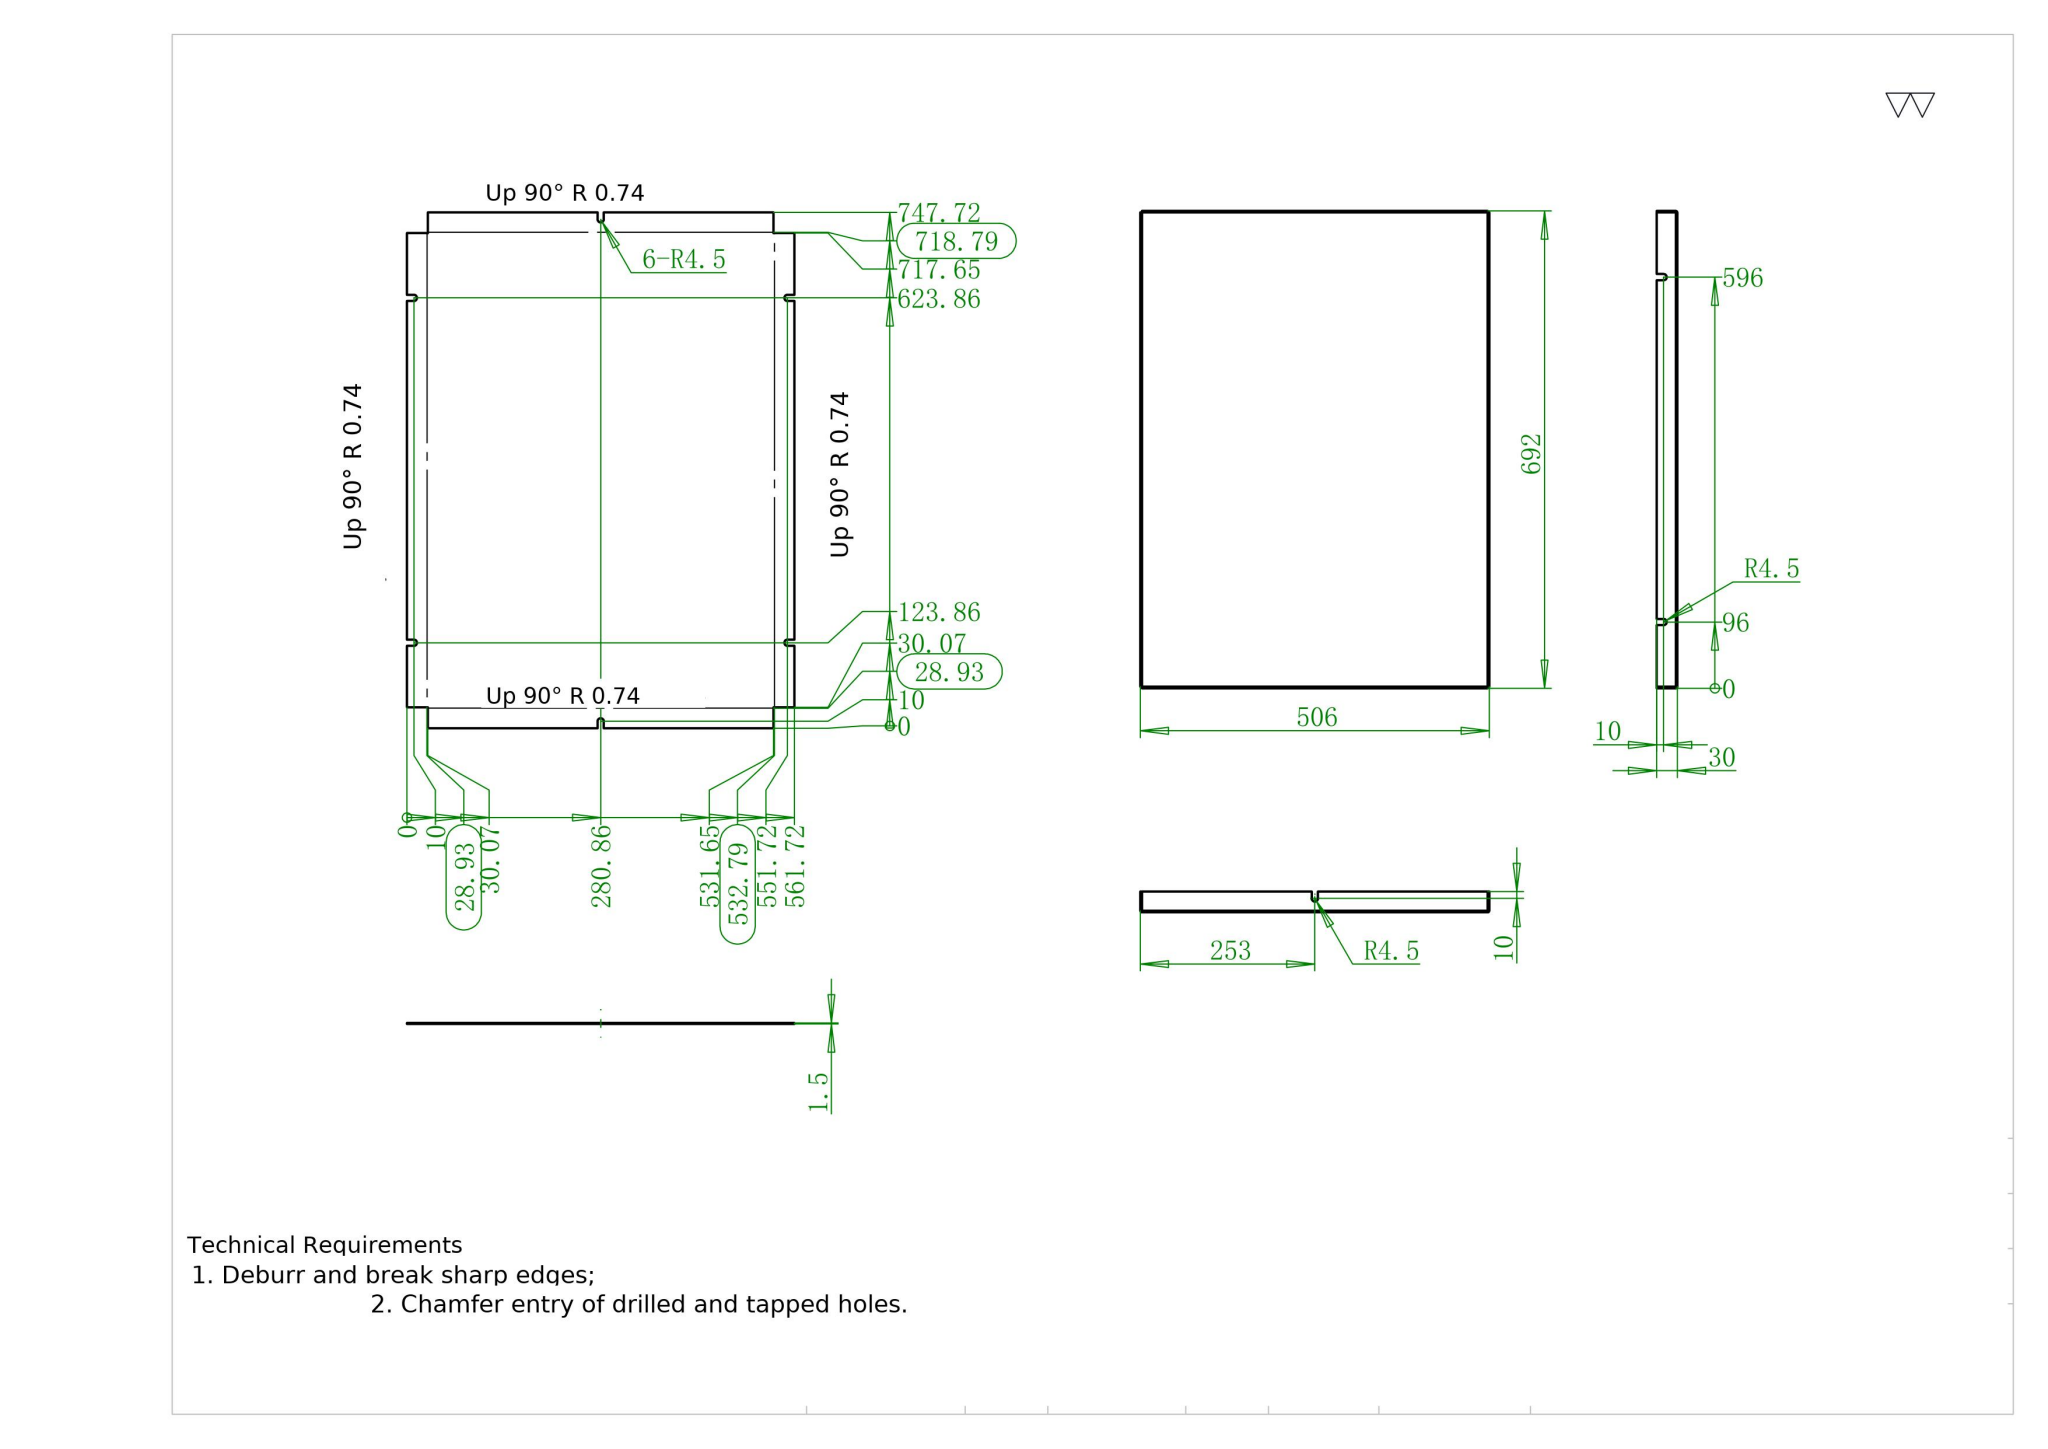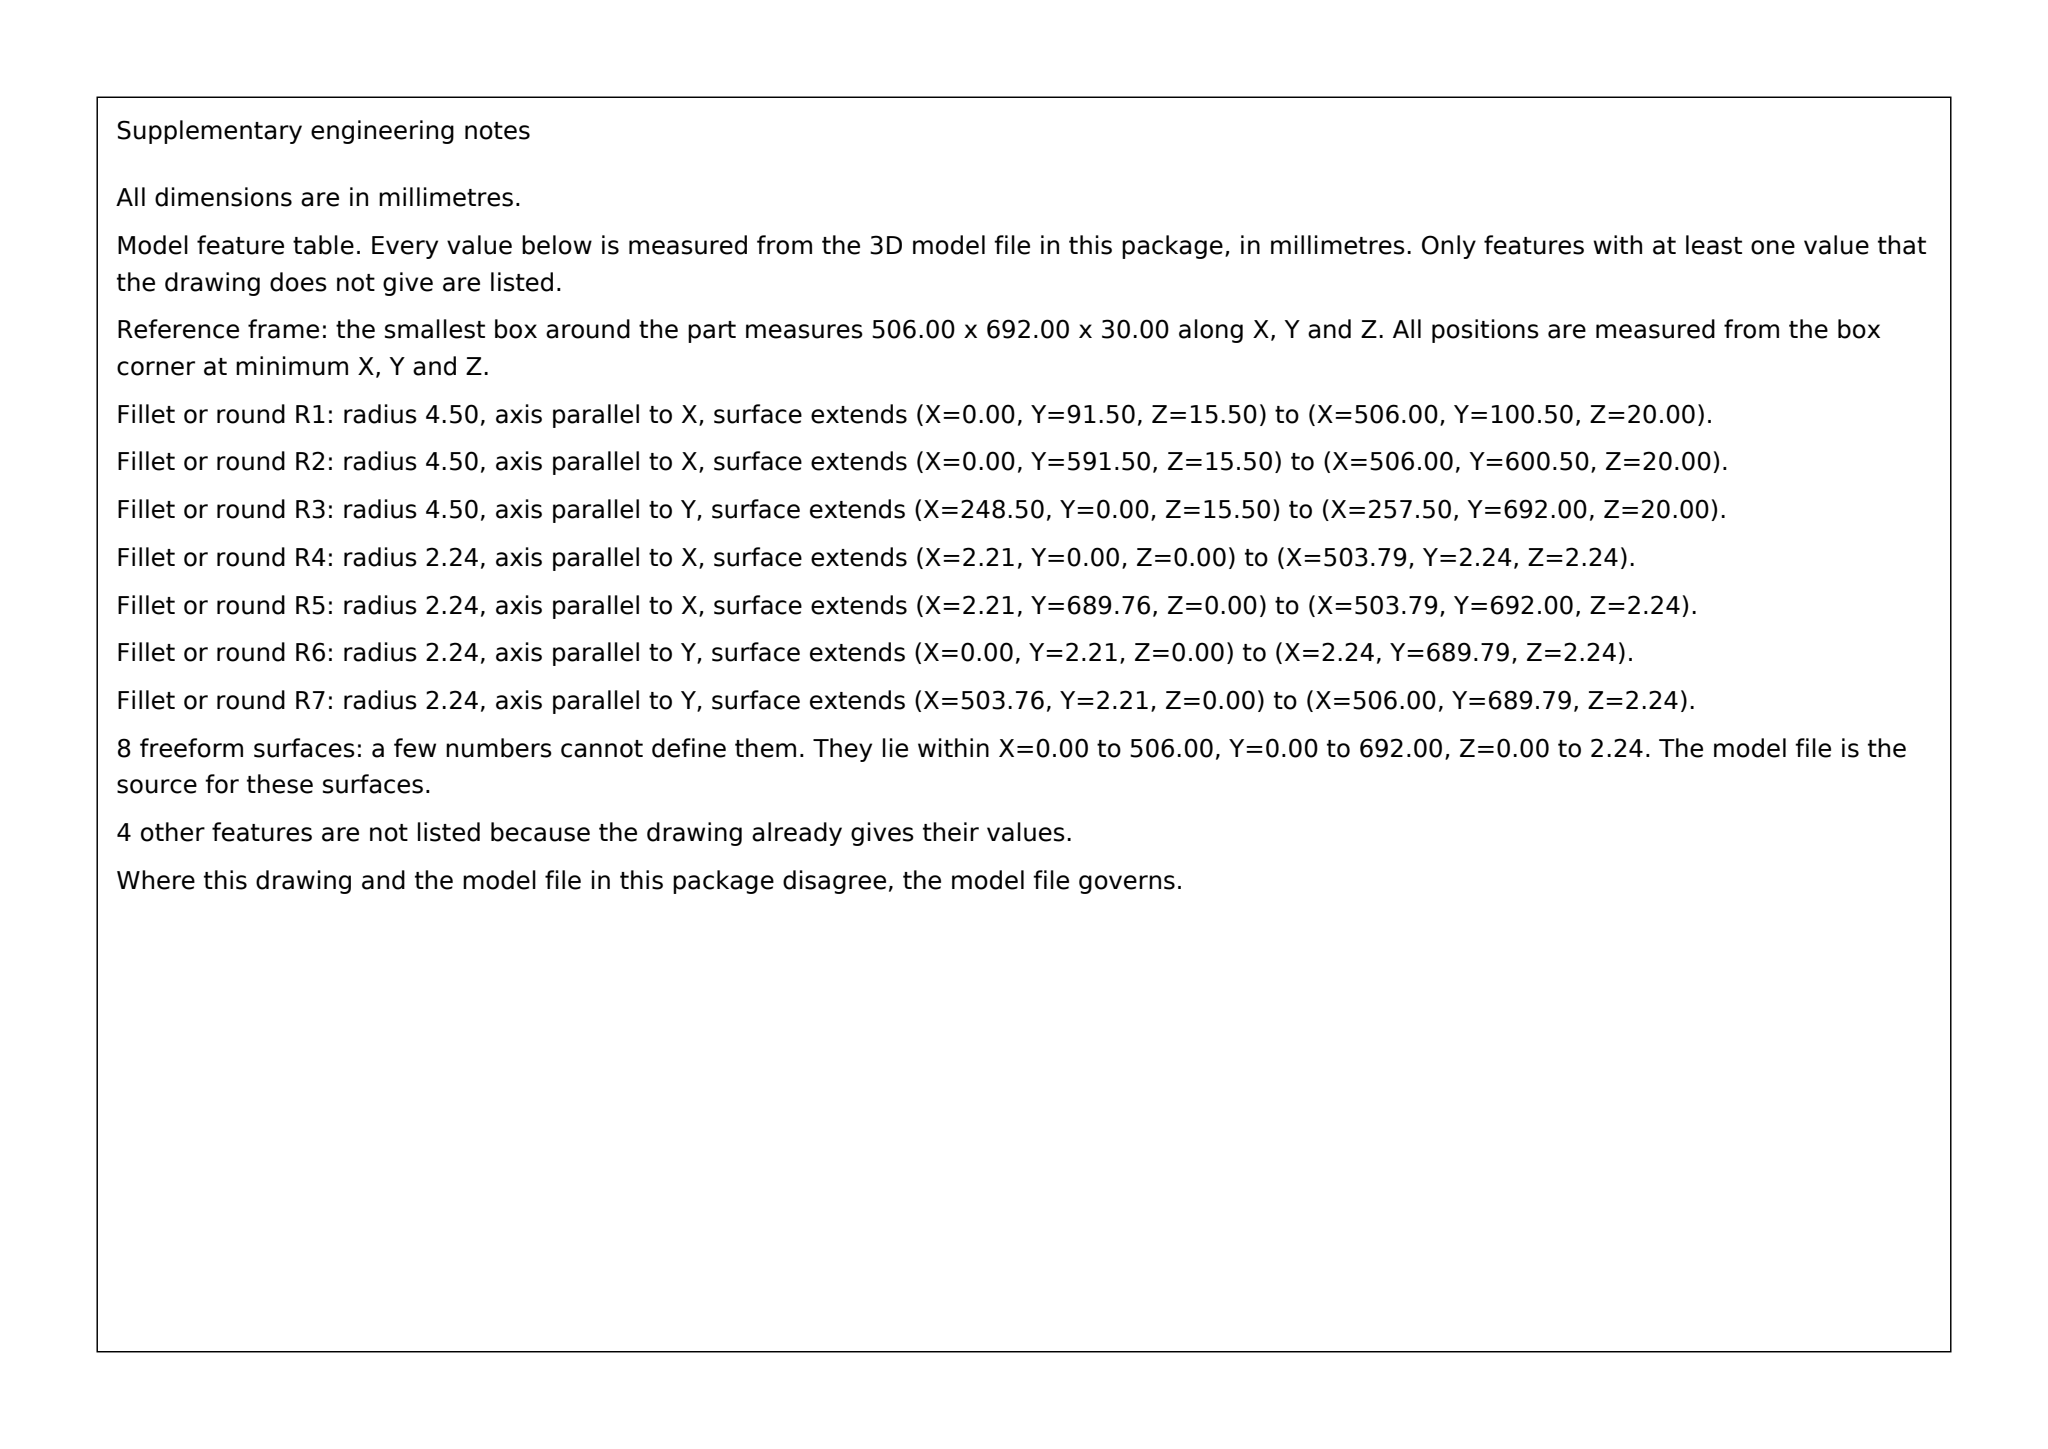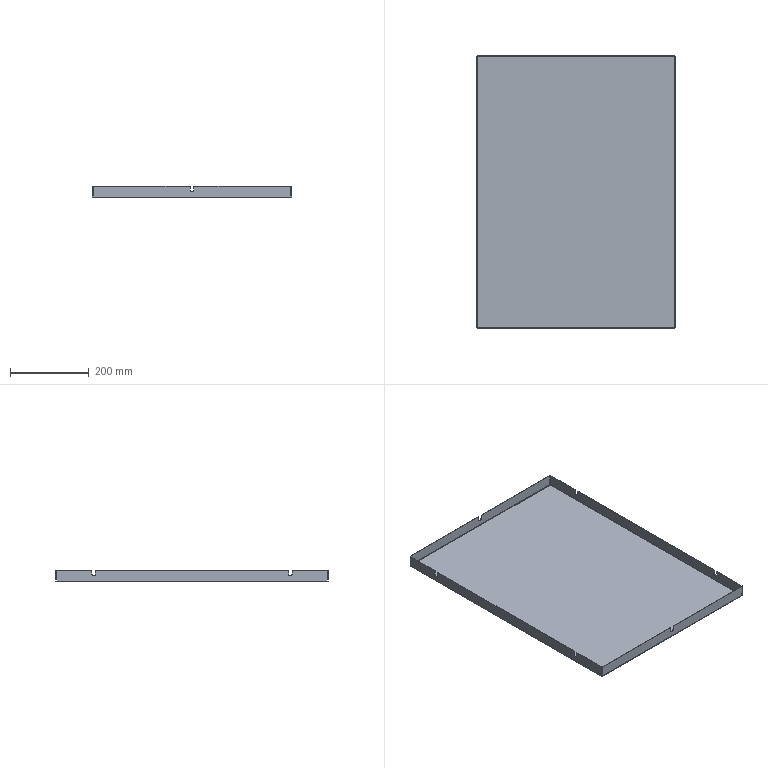Part | SolidWorks | mm | 1 solid | 66 faces | box 506 x 692 x 30 mm | volume 623500 mm3 | plane 40 | cylinder 18 | spline 8 | commonest cylinder face diameters 9 x10 4.473 x4 1.473 x4